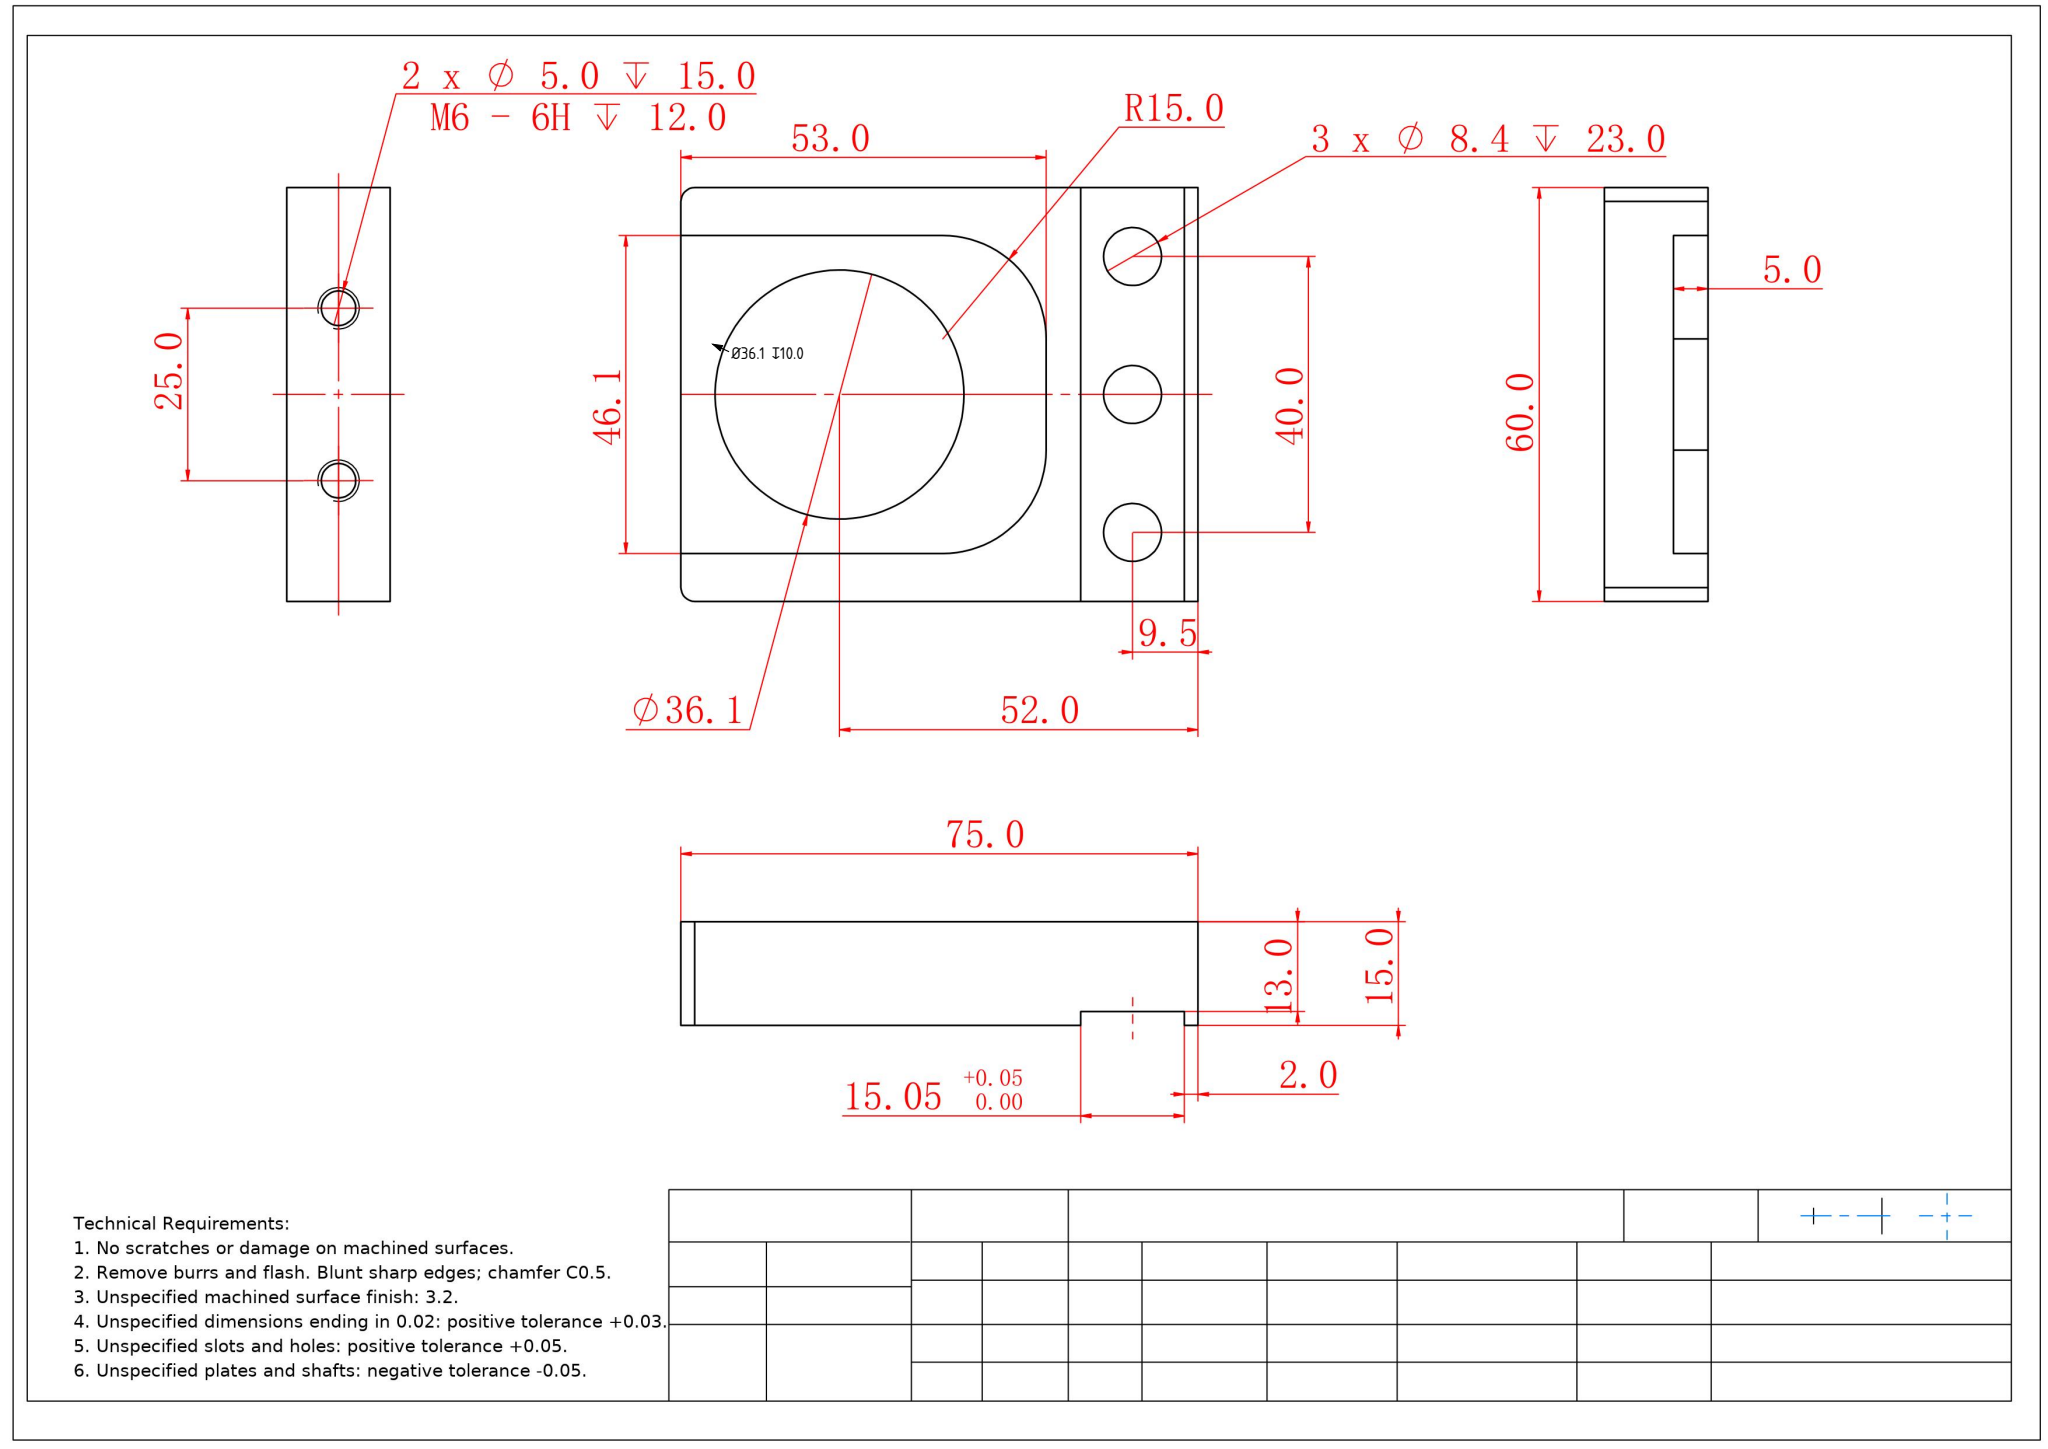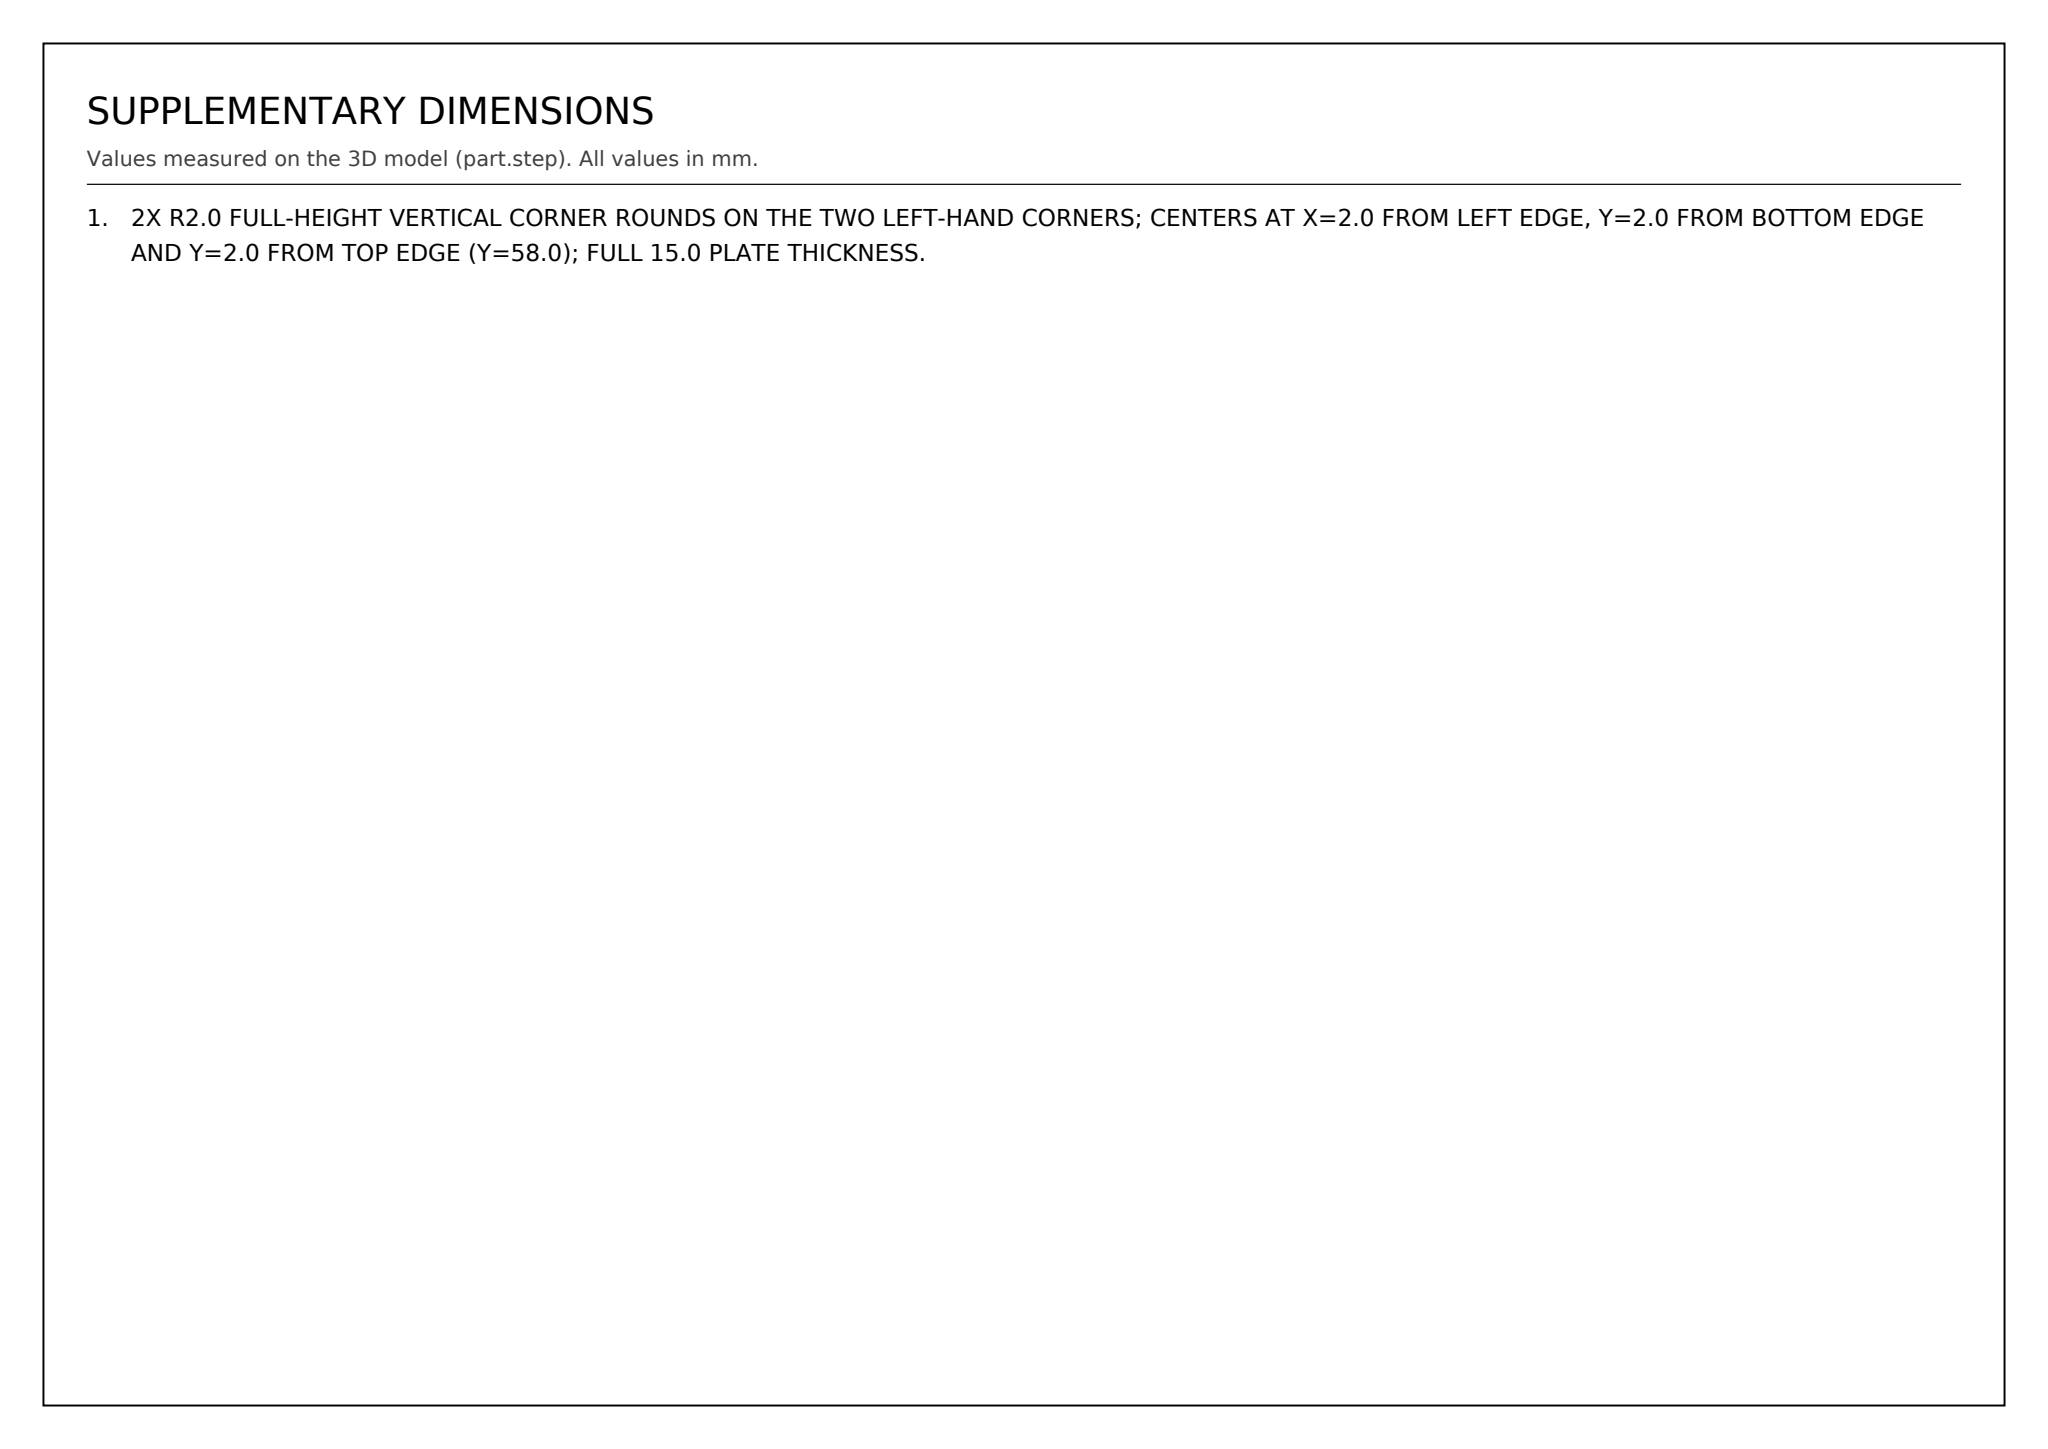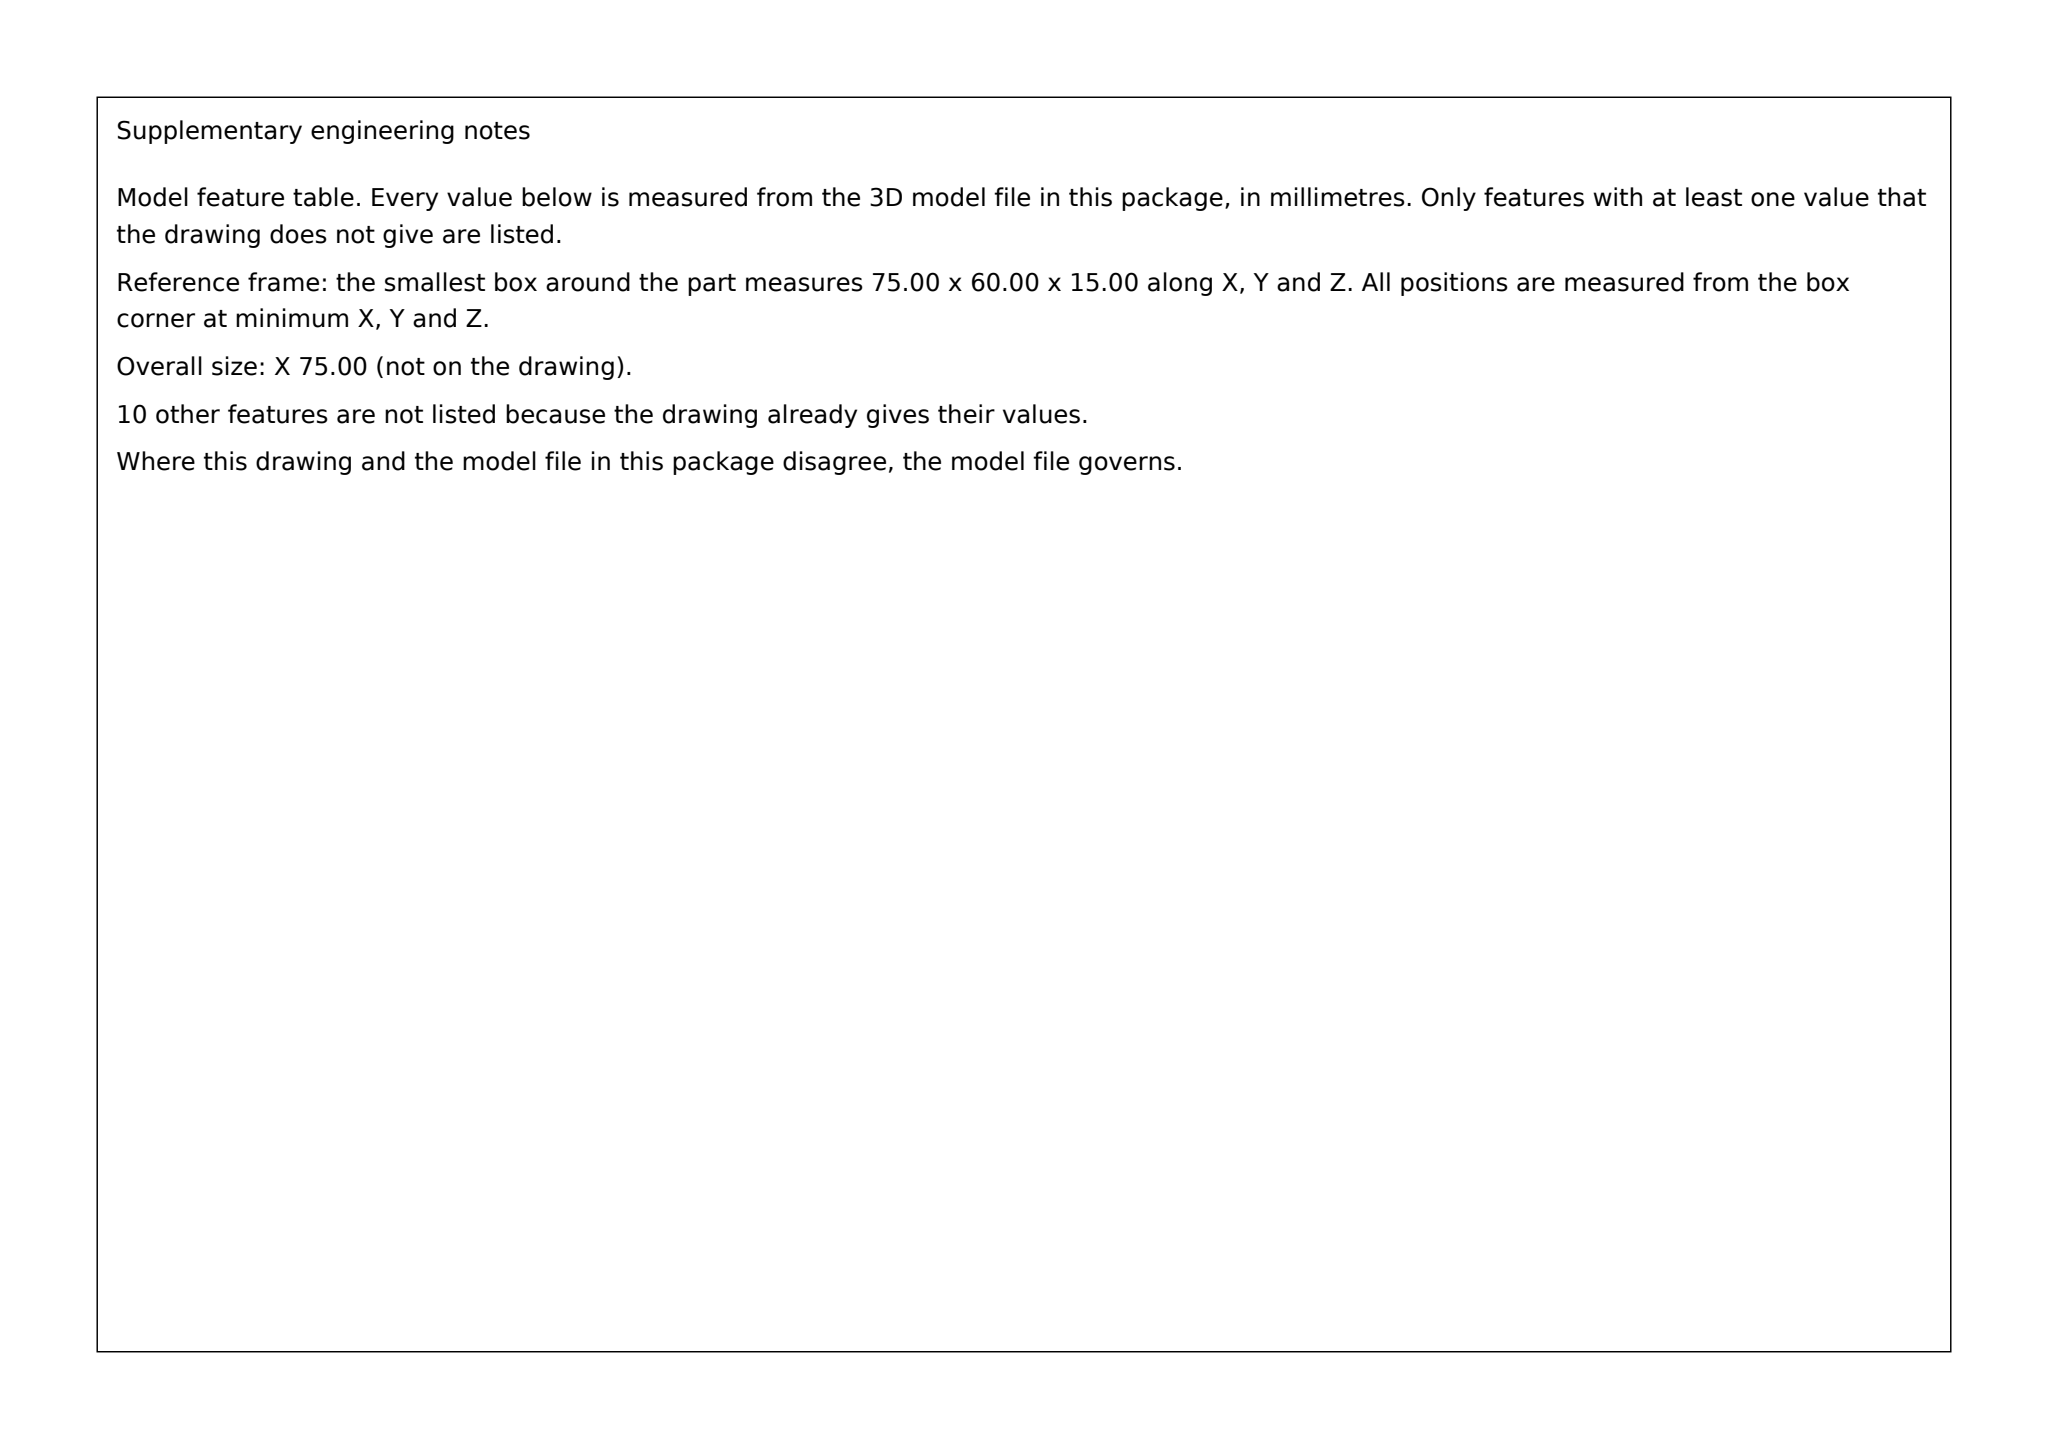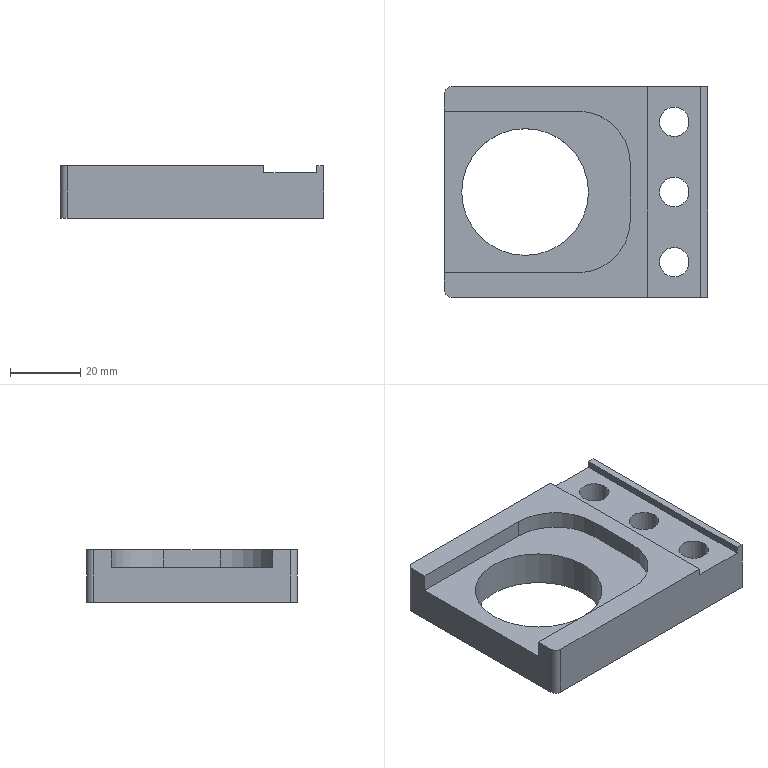Part | SolidWorks | mm | 1 solid | 34 faces | box 75 x 60 x 15 mm | volume 40935 mm3 | cylinder 16 | plane 14 | cone 4 | commonest cylinder face diameters 8.4 x6 5 x4 36.1 x2 30 x2 4 x2
Drawing notes:
Ø36.1 BORE 10.0 DEEP, C/L 23.0 FROM LEFT EDGE AND 30.0 FROM BOTTOM EDGE | from the solid: cylinders entry [36.1, "z", [23.0, 30.0, null], 10.0] and axis plane z=10.0 (bore floor below z=15.0 top face)
2X R2.0 FULL-HEIGHT VERTICAL CORNER ROUNDS ON THE TWO LEFT-HAND CORNERS; CENTERS AT X=2.0 FROM LEFT EDGE, Y=2.0 FROM BOTTOM EDGE AND Y=2.0 FROM TOP EDGE (Y=58.0); FULL 15.0 PLATE THICKNESS. | from the solid: cylinders: two 'convex arc (round/outer radius)' dia 4.0 (R2.0), axis z at [2.0,2.0] and [2.0,58.0], from z=0.0 to z=15.0, arc 90 deg
build123d program:
from build123d import *

# Parameters (mm, degrees)
SKETCH1_W                 = 75
SKETCH1_H                 = 60
BOSS_EXTRUDE1_DEPTH       = 15
SKETCH2_R                 = 18.05
CUT_EXTRUDE1_DEPTH        = 51.312
M8_CLEARANCE_HOLE_1_D     = 8.4
M8_CLEARANCE_HOLE_1_DEPTH = 23
SKETCH10_W                = 15.05
SKETCH10_H                = 60
CUT_EXTRUDE2_DEPTH        = 2
SKETCH11_W                = 65.841
SKETCH11_H                = 46.1
CUT_EXTRUDE3_DEPTH        = 5
FILLET1_R                 = 15
FILLET2_R                 = 2
M6_TAPPED_HOLE1_D         = 5
M6_TAPPED_HOLE1_DEPTH     = 15
M6_TAPPED_HOLE1_TIP       = 1.502


with BuildPart() as part:
    # Sketch1 → Boss-Extrude1 (new body)
    with BuildSketch(Plane.XY):
        Rectangle(SKETCH1_W, SKETCH1_H)
    extrude(amount=BOSS_EXTRUDE1_DEPTH)

    # Sketch2 → Cut-Extrude1 (cut, through all)
    with BuildSketch(Plane.XY.offset(15)):
        with Locations((-14.5, 0)):
            Circle(SKETCH2_R)
    extrude(amount=-CUT_EXTRUDE1_DEPTH, mode=Mode.SUBTRACT)

    # M8 Clearance Hole 1
    with Locations(Plane(origin=(32.5, 0, 0), x_dir=(1, 0, 0), z_dir=(0, 0, -1))):
        with Locations((-4.5, -20), (-4.5, 20), (-4.5, 0)):
            Hole(M8_CLEARANCE_HOLE_1_D / 2, depth=M8_CLEARANCE_HOLE_1_DEPTH)

    # Sketch10 → Cut-Extrude2 (cut)
    with BuildSketch(Plane.XY.offset(15)):
        with Locations((28, 0)):
            Rectangle(SKETCH10_W, SKETCH10_H)
    extrude(amount=-CUT_EXTRUDE2_DEPTH, mode=Mode.SUBTRACT)

    # Sketch11 → Cut-Extrude3 (cut)
    with BuildSketch(Plane.XY.offset(15)):
        with Locations((-17.446, 0)):
            Rectangle(SKETCH11_W, SKETCH11_H)
    extrude(amount=-CUT_EXTRUDE3_DEPTH, mode=Mode.SUBTRACT)

    # Fillet1
    fillet1_edges = [part.edges().sort_by_distance(p)[0] for p in [
        (15.475, -23.05, 12.5),
        (15.475, 23.05, 12.5),
    ]]
    fillet(fillet1_edges, radius=FILLET1_R)

    # Fillet2
    fillet2_edges = [part.edges().sort_by_distance(p)[0] for p in [
        (-37.5, -30, 7.5),
        (-37.5, 30, 7.5),
    ]]
    fillet(fillet2_edges, radius=FILLET2_R)

    # M6 Tapped Hole1
    with Locations(Plane(origin=(37.5, 0, 0), x_dir=(0, 0, -1), z_dir=(1, 0, 0))):
        with Locations((-7.5, 12.5), (-7.5, -12.5)):
            Hole(M6_TAPPED_HOLE1_D / 2, depth=M6_TAPPED_HOLE1_DEPTH)
            with Locations((0, 0, -(M6_TAPPED_HOLE1_DEPTH + M6_TAPPED_HOLE1_TIP / 2))):  # 118° drill point
                Cone(0, M6_TAPPED_HOLE1_D / 2, M6_TAPPED_HOLE1_TIP, mode=Mode.SUBTRACT)


solid = part.part